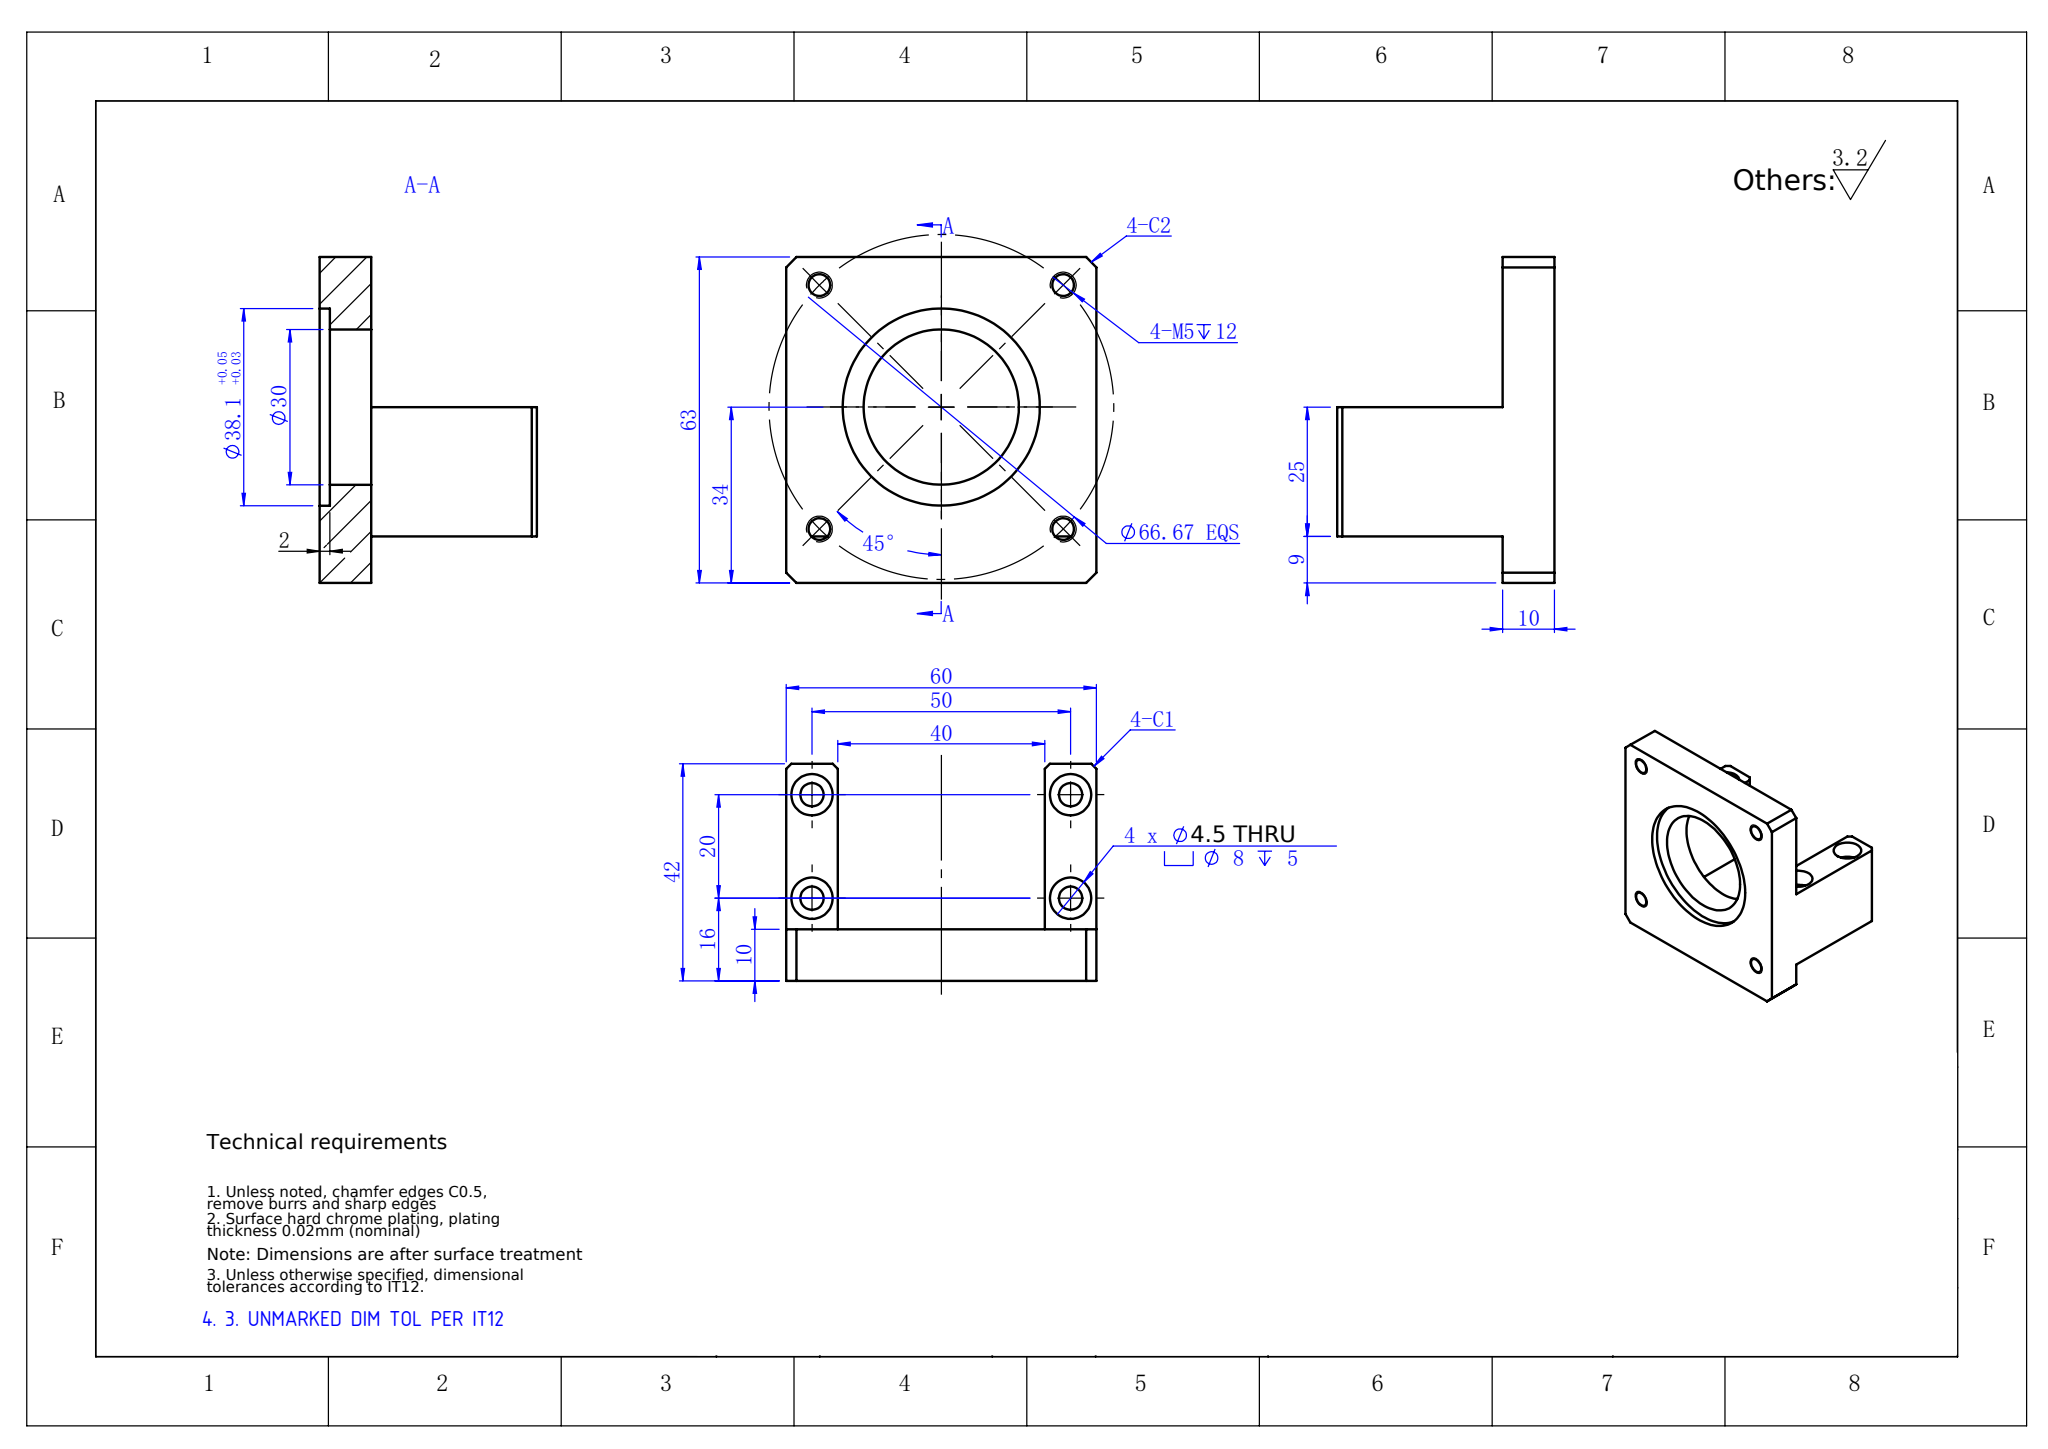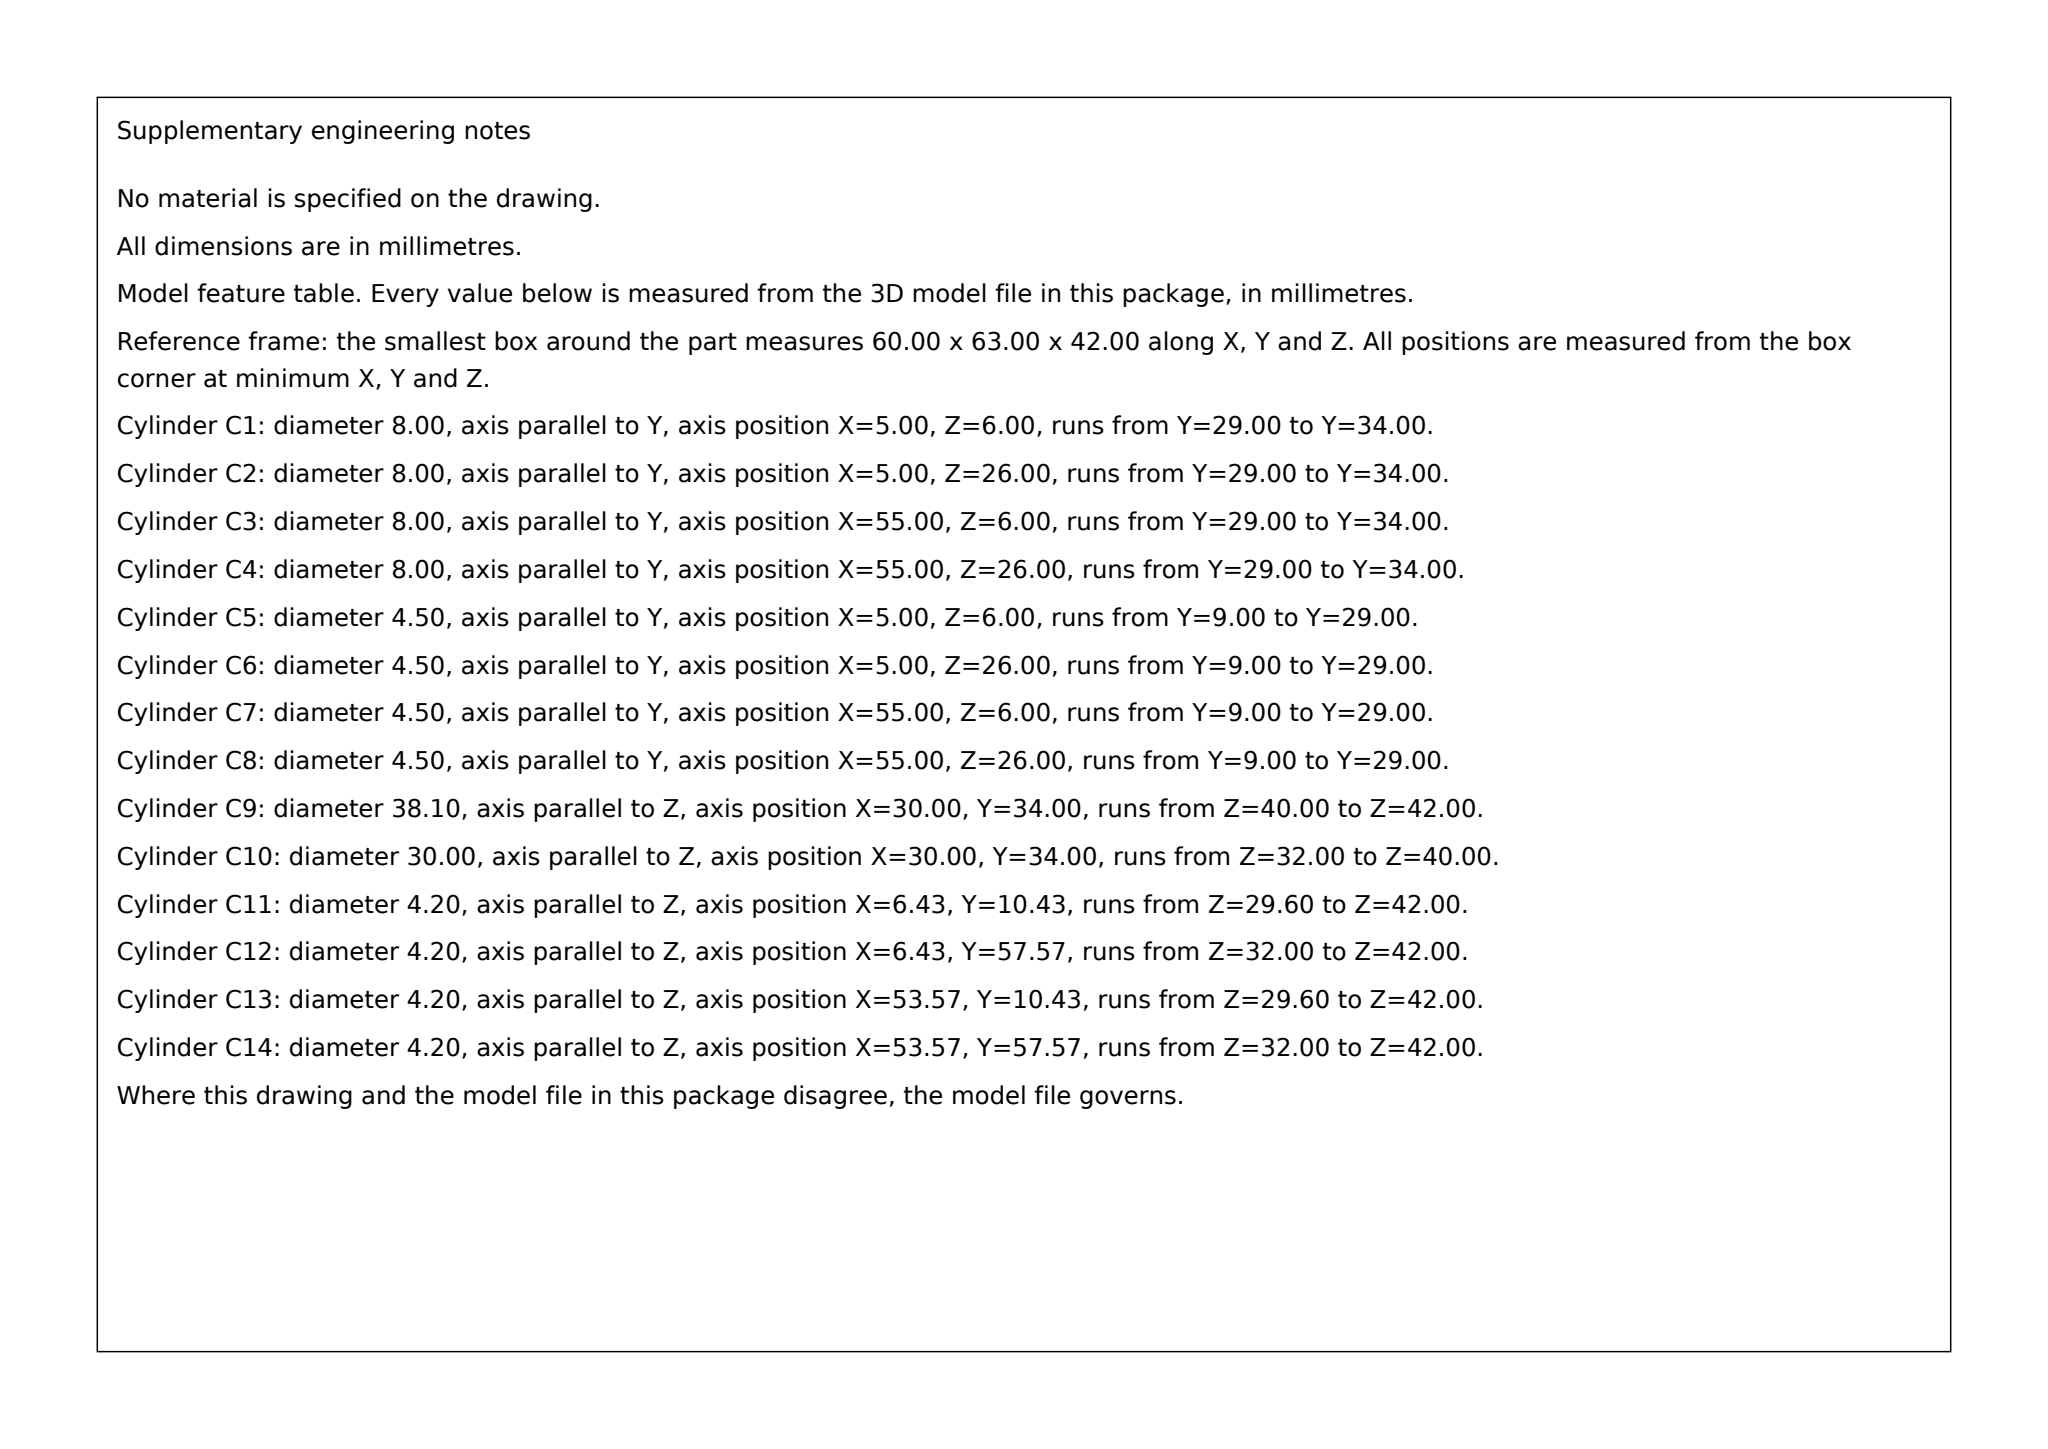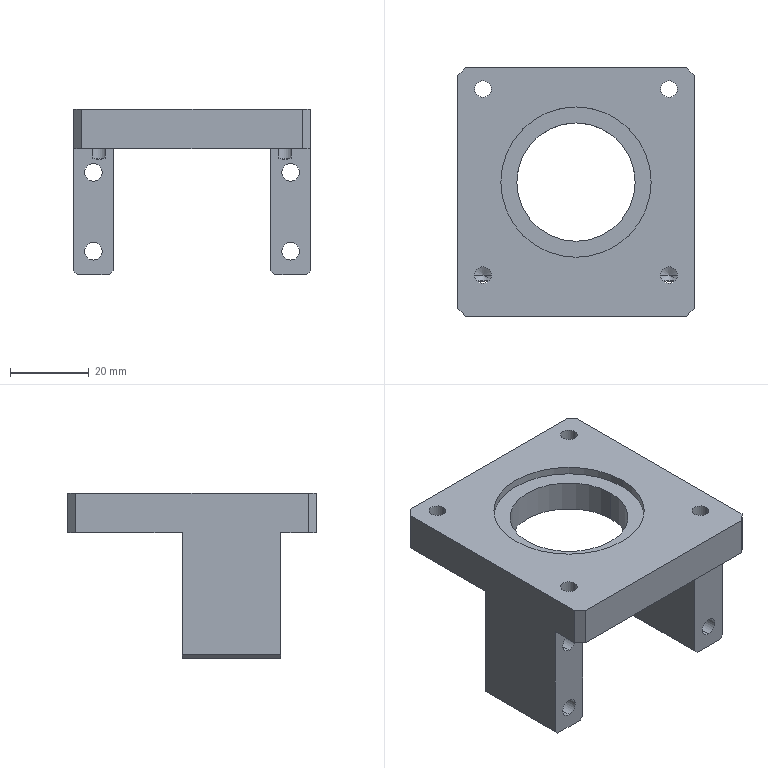Part | SolidWorks | mm | 1 solid | 59 faces | box 60 x 63 x 42 mm | volume 42832 mm3 | cylinder 28 | plane 27 | cone 4 | commonest cylinder face diameters 4.2 x8 8 x8 4.5 x8 38.1 x2 30 x2
Drawing notes:
3. UNMARKED DIM TOL PER IT12 | from the solid: General note; no per-feature tols in STEP (all dims nominal, e.g. 60x63x42 bbox)
build123d program:
from build123d import *

# Parameters (mm, degrees)
BOSS_EXTRUDE4_DEPTH                       = 63
SKETCH6_W                                 = 32
SKETCH6_H                                 = 29
SKETCH6_H_2                               = 9
CUT_EXTRUDE1_DEPTH                        = 55
M4_HEX_HEAD_BOLT_COUNTERBORE1_D           = 4.5
M4_HEX_HEAD_BOLT_COUNTERBORE1_CBORE_D     = 8
M4_HEX_HEAD_BOLT_COUNTERBORE1_CBORE_DEPTH = 5
M5_TAPPED_HOLE1_D                         = 4.2
M5_TAPPED_HOLE1_DEPTH                     = 12.4
M5_TAPPED_HOLE1_TIP                       = 1.262
CHAMFER1_SIZE                             = 2
CHAMFER2_SIZE                             = 1


with BuildPart() as part:
    # Sketch4 → Boss-Extrude4 (new body)
    with BuildSketch(Plane(origin=(0, 0, 0), x_dir=(1, 0, 0), z_dir=(0, 1, 0))):
        Polygon((-30, 0), (30, 0), (30, 42), (20, 42), (20, 10), (-20, 10), (-20, 42), (-30, 42), align=None)
    extrude(amount=BOSS_EXTRUDE4_DEPTH)

    # Sketch5 → Cut-Revolve1 (revolve, cut)
    with BuildSketch(Plane(origin=(0, 0, 0), x_dir=(0, 0, -1), z_dir=(1, 0, 0)), mode=Mode.PRIVATE) as cut_revolve1_sk:
        Polygon((0, 53.05), (2, 53.05), (2, 49), (42, 49), (42, 34), (0, 34), align=None)
    revolve(cut_revolve1_sk.sketch.rotate(Axis((0, 34, 16.806), (0, 0, -1)), 90), axis=Axis((0, 34, 16.806), (0, 0, -1)), mode=Mode.SUBTRACT)

    # Sketch6 → Cut-Extrude1 (cut, symmetric)
    with BuildSketch(Plane(origin=(0, 0, 0), x_dir=(0, 0, -1), z_dir=(1, 0, 0))):
        with Locations((26, 48.5)):
            Rectangle(SKETCH6_W, SKETCH6_H)
        with Locations((26, 4.5)):
            Rectangle(SKETCH6_W, SKETCH6_H_2)
    extrude(amount=CUT_EXTRUDE1_DEPTH, both=True, mode=Mode.SUBTRACT)

    # M4 Hex Head Bolt Counterbore1 (through all)
    with Locations(Plane(origin=(0, 34, 0), x_dir=(1, 0, 0), z_dir=(0, 1, 0))):
        with Locations((-25, 36), (-25, 16), (25, 36), (25, 16)):
            CounterBoreHole(M4_HEX_HEAD_BOLT_COUNTERBORE1_D / 2, M4_HEX_HEAD_BOLT_COUNTERBORE1_CBORE_D / 2, M4_HEX_HEAD_BOLT_COUNTERBORE1_CBORE_DEPTH)

    # M5 Tapped Hole1
    with Locations(Plane.XY):
        with Locations((-23.571, 57.571), (23.571, 57.571), (23.571, 10.429), (-23.571, 10.429)):
            Hole(M5_TAPPED_HOLE1_D / 2, depth=M5_TAPPED_HOLE1_DEPTH)
            with Locations((0, 0, -(M5_TAPPED_HOLE1_DEPTH + M5_TAPPED_HOLE1_TIP / 2))):  # 118° drill point
                Cone(0, M5_TAPPED_HOLE1_D / 2, M5_TAPPED_HOLE1_TIP, mode=Mode.SUBTRACT)

    # Chamfer1
    chamfer1_edges = [part.edges().sort_by_distance(p)[0] for p in [
        (30, 63, -5),
        (-30, 63, -5),
        (-30, 0, -5),
        (30, 0, -5),
    ]]
    chamfer(chamfer1_edges, length=CHAMFER1_SIZE)

    # Chamfer2
    chamfer2_edges = [part.edges().sort_by_distance(p)[0] for p in [
        (-30, 21.5, -42),
        (-20, 21.5, -42),
        (20, 21.5, -42),
        (30, 21.5, -42),
    ]]
    chamfer(chamfer2_edges, length=CHAMFER2_SIZE)


solid = part.part